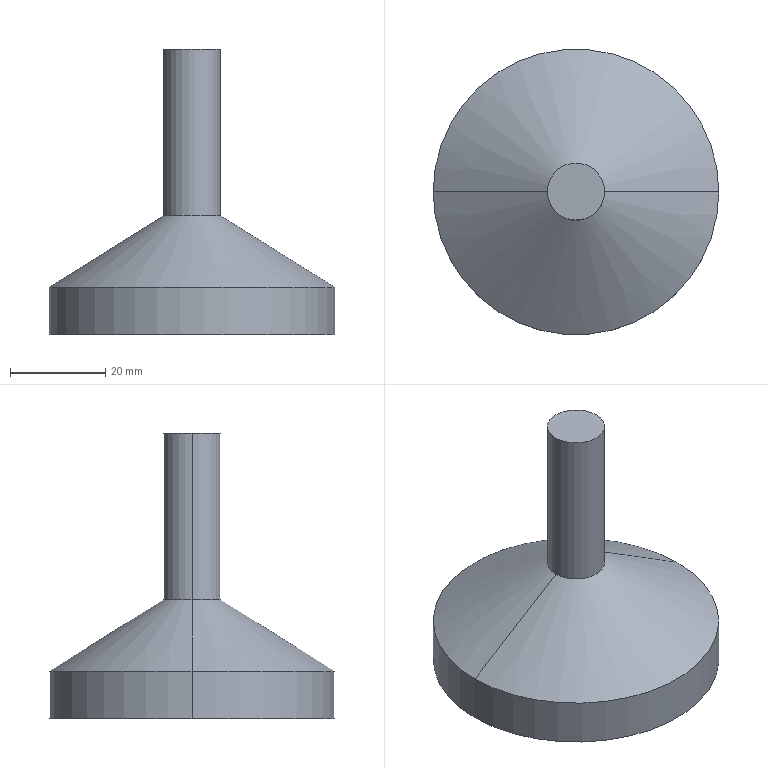Component | SolidWorks | FootPad-1 | 1 solid | 8 faces | box 60 x 60 x 60 mm | volume 49763 mm3 | cylinder 4 | cone 2 | plane 2 | commonest cylinder face diameters 60 x2 12 x2 | material Stainless Steel (Ferritic)
build123d program:
from build123d import *


with BuildPart() as part:
    # Sketch1 → Revolve1 (revolve)
    with BuildSketch(Plane(origin=(0, 0, 0), x_dir=(0, 0, -1), z_dir=(1, 0, 0)), mode=Mode.PRIVATE) as revolve1_sk:
        Polygon((0, 60), (-6, 60), (-6, 25), (-30, 10), (-30, 0), (0, 0), align=None)
    revolve(revolve1_sk.sketch.rotate(Axis((0, 0, 0), (0, 1, 0)), 180), axis=Axis((0, 0, 0), (0, 1, 0)))


solid = part.part

# Placed as in the assembly
solid = solid.moved(Location((1315.186, 858.312, 1361.454), (90, 0, 0)))
STEP:
#1=CARTESIAN_POINT('',(50.598,33.792,53.994));
#2=VERTEX_POINT('',#1);
#3=CARTESIAN_POINT('',(52.96,33.792,53.994));
#4=VERTEX_POINT('',#3);
#5=CARTESIAN_POINT('',(51.779,33.792,53.994));
#6=DIRECTION('',(-0.,0.,-1.));
#7=DIRECTION('',(-1.,0.,0.));
#8=AXIS2_PLACEMENT_3D('',#5,#6,#7);
#9=CIRCLE('',#8,1.181);
#10=EDGE_CURVE('',#2,#4,#9,.T.);
#11=ORIENTED_EDGE('',*,*,#10,.T.);
#12=CARTESIAN_POINT('',(52.96,33.792,53.601));
#13=VERTEX_POINT('',#12);
#14=CARTESIAN_POINT('',(52.96,33.792,53.601));
#15=DIRECTION('',(-0.,0.,-1.));
#16=VECTOR('',#15,39.37);
#17=LINE('',#14,#16);
#18=EDGE_CURVE('',#4,#13,#17,.T.);
#19=ORIENTED_EDGE('',*,*,#18,.T.);
#20=CARTESIAN_POINT('',(50.598,33.792,53.601));
#21=VERTEX_POINT('',#20);
#22=CARTESIAN_POINT('',(51.779,33.792,53.601));
#23=DIRECTION('',(-0.,0.,-1.));
#24=DIRECTION('',(-1.,0.,0.));
#25=AXIS2_PLACEMENT_3D('',#22,#23,#24);
#26=CIRCLE('',#25,1.181);
#27=EDGE_CURVE('',#21,#13,#26,.T.);
#28=ORIENTED_EDGE('',*,*,#27,.F.);
#29=CARTESIAN_POINT('',(50.598,33.792,53.601));
#30=DIRECTION('',(-0.,0.,-1.));
#31=VECTOR('',#30,39.37);
#32=LINE('',#29,#31);
#33=EDGE_CURVE('',#2,#21,#32,.T.);
#34=ORIENTED_EDGE('',*,*,#33,.F.);
#35=EDGE_LOOP('',(#11,#19,#28,#34));
#36=FACE_OUTER_BOUND('',#35,.T.);
#37=CARTESIAN_POINT('',(51.779,33.792,53.601));
#38=DIRECTION('',(-0.,0.,-1.));
#39=DIRECTION('',(-1.,0.,0.));
#40=AXIS2_PLACEMENT_3D('',#37,#38,#39);
#41=CYLINDRICAL_SURFACE('',#40,1.181);
#42=ADVANCED_FACE('',(#36),#41,.T.);
#43=CARTESIAN_POINT('',(51.543,33.792,54.585));
#44=VERTEX_POINT('',#43);
#45=CARTESIAN_POINT('',(52.015,33.792,54.585));
#46=VERTEX_POINT('',#45);
#47=CARTESIAN_POINT('',(51.779,33.792,54.585));
#48=DIRECTION('',(-0.,0.,-1.));
#49=DIRECTION('',(-1.,0.,0.));
#50=AXIS2_PLACEMENT_3D('',#47,#48,#49);
#51=CIRCLE('',#50,0.2362);
#52=EDGE_CURVE('',#44,#46,#51,.T.);
#53=ORIENTED_EDGE('',*,*,#52,.T.);
#54=CARTESIAN_POINT('',(52.015,33.792,54.585));
#55=DIRECTION('',(0.848,0.,-0.53));
#56=VECTOR('',#55,39.37);
#57=LINE('',#54,#56);
#58=EDGE_CURVE('',#46,#4,#57,.T.);
#59=ORIENTED_EDGE('',*,*,#58,.T.);
#60=ORIENTED_EDGE('',*,*,#10,.F.);
#61=CARTESIAN_POINT('',(51.543,33.792,54.585));
#62=DIRECTION('',(-0.848,0.,-0.53));
#63=VECTOR('',#62,39.37);
#64=LINE('',#61,#63);
#65=EDGE_CURVE('',#44,#2,#64,.T.);
#66=ORIENTED_EDGE('',*,*,#65,.F.);
#67=EDGE_LOOP('',(#53,#59,#60,#66));
#68=FACE_OUTER_BOUND('',#67,.T.);
#69=CARTESIAN_POINT('',(51.779,33.792,54.585));
#70=DIRECTION('',(-0.,0.,-1.));
#71=DIRECTION('',(-1.,0.,0.));
#72=AXIS2_PLACEMENT_3D('',#69,#70,#71);
#73=CONICAL_SURFACE('',#72,0.2362,1.012);
#74=ADVANCED_FACE('',(#68),#73,.T.);
#75=CARTESIAN_POINT('',(51.543,33.792,55.963));
#76=VERTEX_POINT('',#75);
#77=CARTESIAN_POINT('',(52.015,33.792,55.963));
#78=VERTEX_POINT('',#77);
#79=CARTESIAN_POINT('',(51.779,33.792,55.963));
#80=DIRECTION('',(-0.,0.,-1.));
#81=DIRECTION('',(-1.,0.,0.));
#82=AXIS2_PLACEMENT_3D('',#79,#80,#81);
#83=CIRCLE('',#82,0.2362);
#84=EDGE_CURVE('',#76,#78,#83,.T.);
#85=ORIENTED_EDGE('',*,*,#84,.T.);
#86=CARTESIAN_POINT('',(52.015,33.792,53.601));
#87=DIRECTION('',(-0.,0.,-1.));
#88=VECTOR('',#87,39.37);
#89=LINE('',#86,#88);
#90=EDGE_CURVE('',#78,#46,#89,.T.);
#91=ORIENTED_EDGE('',*,*,#90,.T.);
#92=ORIENTED_EDGE('',*,*,#52,.F.);
#93=CARTESIAN_POINT('',(51.543,33.792,53.601));
#94=DIRECTION('',(-0.,0.,-1.));
#95=VECTOR('',#94,39.37);
#96=LINE('',#93,#95);
#97=EDGE_CURVE('',#76,#44,#96,.T.);
#98=ORIENTED_EDGE('',*,*,#97,.F.);
#99=EDGE_LOOP('',(#85,#91,#92,#98));
#100=FACE_OUTER_BOUND('',#99,.T.);
#101=CARTESIAN_POINT('',(51.779,33.792,53.601));
#102=DIRECTION('',(-0.,0.,-1.));
#103=DIRECTION('',(-1.,0.,0.));
#104=AXIS2_PLACEMENT_3D('',#101,#102,#103);
#105=CYLINDRICAL_SURFACE('',#104,0.2362);
#106=ADVANCED_FACE('',(#100),#105,.T.);
#107=ORIENTED_EDGE('',*,*,#84,.F.);
#108=CARTESIAN_POINT('',(51.779,33.792,55.963));
#109=DIRECTION('',(-0.,0.,-1.));
#110=DIRECTION('',(-1.,0.,0.));
#111=AXIS2_PLACEMENT_3D('',#108,#109,#110);
#112=CIRCLE('',#111,0.2362);
#113=EDGE_CURVE('',#78,#76,#112,.T.);
#114=ORIENTED_EDGE('',*,*,#113,.F.);
#115=EDGE_LOOP('',(#107,#114));
#116=FACE_OUTER_BOUND('',#115,.T.);
#117=CARTESIAN_POINT('',(51.779,33.792,55.963));
#118=DIRECTION('',(-0.,0.,-1.));
#119=DIRECTION('',(-1.,0.,0.));
#120=AXIS2_PLACEMENT_3D('',#117,#118,#119);
#121=PLANE('',#120);
#122=ADVANCED_FACE('',(#116),#121,.F.);
#123=ORIENTED_EDGE('',*,*,#90,.F.);
#124=ORIENTED_EDGE('',*,*,#113,.T.);
#125=ORIENTED_EDGE('',*,*,#97,.T.);
#126=CARTESIAN_POINT('',(51.779,33.792,54.585));
#127=DIRECTION('',(-0.,0.,-1.));
#128=DIRECTION('',(-1.,0.,0.));
#129=AXIS2_PLACEMENT_3D('',#126,#127,#128);
#130=CIRCLE('',#129,0.2362);
#131=EDGE_CURVE('',#46,#44,#130,.T.);
#132=ORIENTED_EDGE('',*,*,#131,.F.);
#133=EDGE_LOOP('',(#123,#124,#125,#132));
#134=FACE_OUTER_BOUND('',#133,.T.);
#135=CARTESIAN_POINT('',(51.779,33.792,53.601));
#136=DIRECTION('',(-0.,0.,-1.));
#137=DIRECTION('',(-1.,0.,0.));
#138=AXIS2_PLACEMENT_3D('',#135,#136,#137);
#139=CYLINDRICAL_SURFACE('',#138,0.2362);
#140=ADVANCED_FACE('',(#134),#139,.T.);
#141=ORIENTED_EDGE('',*,*,#58,.F.);
#142=ORIENTED_EDGE('',*,*,#131,.T.);
#143=ORIENTED_EDGE('',*,*,#65,.T.);
#144=CARTESIAN_POINT('',(51.779,33.792,53.994));
#145=DIRECTION('',(-0.,0.,-1.));
#146=DIRECTION('',(-1.,0.,0.));
#147=AXIS2_PLACEMENT_3D('',#144,#145,#146);
#148=CIRCLE('',#147,1.181);
#149=EDGE_CURVE('',#4,#2,#148,.T.);
#150=ORIENTED_EDGE('',*,*,#149,.F.);
#151=EDGE_LOOP('',(#141,#142,#143,#150));
#152=FACE_OUTER_BOUND('',#151,.T.);
#153=CARTESIAN_POINT('',(51.779,33.792,54.585));
#154=DIRECTION('',(-0.,0.,-1.));
#155=DIRECTION('',(-1.,0.,0.));
#156=AXIS2_PLACEMENT_3D('',#153,#154,#155);
#157=CONICAL_SURFACE('',#156,0.2362,1.012);
#158=ADVANCED_FACE('',(#152),#157,.T.);
#159=ORIENTED_EDGE('',*,*,#18,.F.);
#160=ORIENTED_EDGE('',*,*,#149,.T.);
#161=ORIENTED_EDGE('',*,*,#33,.T.);
#162=CARTESIAN_POINT('',(51.779,33.792,53.601));
#163=DIRECTION('',(-0.,0.,-1.));
#164=DIRECTION('',(-1.,0.,0.));
#165=AXIS2_PLACEMENT_3D('',#162,#163,#164);
#166=CIRCLE('',#165,1.181);
#167=EDGE_CURVE('',#13,#21,#166,.T.);
#168=ORIENTED_EDGE('',*,*,#167,.F.);
#169=EDGE_LOOP('',(#159,#160,#161,#168));
#170=FACE_OUTER_BOUND('',#169,.T.);
#171=CARTESIAN_POINT('',(51.779,33.792,53.601));
#172=DIRECTION('',(-0.,0.,-1.));
#173=DIRECTION('',(-1.,0.,0.));
#174=AXIS2_PLACEMENT_3D('',#171,#172,#173);
#175=CYLINDRICAL_SURFACE('',#174,1.181);
#176=ADVANCED_FACE('',(#170),#175,.T.);
#177=ORIENTED_EDGE('',*,*,#27,.T.);
#178=ORIENTED_EDGE('',*,*,#167,.T.);
#179=EDGE_LOOP('',(#177,#178));
#180=FACE_OUTER_BOUND('',#179,.T.);
#181=CARTESIAN_POINT('',(52.96,33.792,53.601));
#182=DIRECTION('',(0.,-0.,1.));
#183=DIRECTION('',(1.,0.,-0.));
#184=AXIS2_PLACEMENT_3D('',#181,#182,#183);
#185=PLANE('',#184);
#186=ADVANCED_FACE('',(#180),#185,.F.);
#187=CLOSED_SHELL('',(#42,#74,#106,#122,#140,#158,#176,#186));
#188=MANIFOLD_SOLID_BREP('',#187);
#189=CARTESIAN_POINT('',(0.,0.,0.));
#190=DIRECTION('',(0.,0.,1.));
#191=DIRECTION('',(1.,0.,0.));
#192=AXIS2_PLACEMENT_3D('',#189,#190,#191);
#193=(LENGTH_UNIT()NAMED_UNIT(*)SI_UNIT($,.METRE.));
#194=LENGTH_MEASURE_WITH_UNIT(LENGTH_MEASURE(0.0254),#193);
#195=DIMENSIONAL_EXPONENTS(1.,0.,0.,0.,0.,0.,0.);
#196=(CONVERSION_BASED_UNIT('',#194)LENGTH_UNIT()NAMED_UNIT(#195));
#197=UNCERTAINTY_MEASURE_WITH_UNIT(LENGTH_MEASURE(0.00001),#196,'','');
#198=(NAMED_UNIT(*)PLANE_ANGLE_UNIT()SI_UNIT($,.RADIAN.));
#199=(NAMED_UNIT(*)SI_UNIT($,.STERADIAN.)SOLID_ANGLE_UNIT());
#200=(GEOMETRIC_REPRESENTATION_CONTEXT(3)GLOBAL_UNCERTAINTY_ASSIGNED_CONTEXT((#197))GLOBAL_UNIT_ASSIGNED_CONTEXT((#196,#198,#199))REPRESENTATION_CONTEXT('',''));
#201=ADVANCED_BREP_SHAPE_REPRESENTATION('',(#188,#192),#200);
#202=COLOUR_RGB('',0.7922,0.8196,0.9333);
#203=FILL_AREA_STYLE_COLOUR('',#202);
#204=FILL_AREA_STYLE('',(#203));
#205=SURFACE_STYLE_FILL_AREA(#204);
#206=SURFACE_SIDE_STYLE('',(#205));
#207=SURFACE_STYLE_USAGE(.BOTH.,#206);
#208=PRESENTATION_STYLE_ASSIGNMENT((#207));
#209=STYLED_ITEM('',(#208),#188);
#210=(LENGTH_UNIT()NAMED_UNIT(*)SI_UNIT($,.METRE.));
#211=LENGTH_MEASURE_WITH_UNIT(LENGTH_MEASURE(0.0254),#210);
#212=DIMENSIONAL_EXPONENTS(1.,0.,0.,0.,0.,0.,0.);
#213=(CONVERSION_BASED_UNIT('',#211)LENGTH_UNIT()NAMED_UNIT(#212));
#214=UNCERTAINTY_MEASURE_WITH_UNIT(LENGTH_MEASURE(0.00001),#213,'','');
#215=(NAMED_UNIT(*)PLANE_ANGLE_UNIT()SI_UNIT($,.RADIAN.));
#216=(NAMED_UNIT(*)SI_UNIT($,.STERADIAN.)SOLID_ANGLE_UNIT());
#217=(GEOMETRIC_REPRESENTATION_CONTEXT(3)GLOBAL_UNCERTAINTY_ASSIGNED_CONTEXT((#214))GLOBAL_UNIT_ASSIGNED_CONTEXT((#213,#215,#216))REPRESENTATION_CONTEXT('',''));
#218=MECHANICAL_DESIGN_GEOMETRIC_PRESENTATION_REPRESENTATION('',(#209),#217);
#219=PRESENTATION_LAYER_ASSIGNMENT('','',(#209));